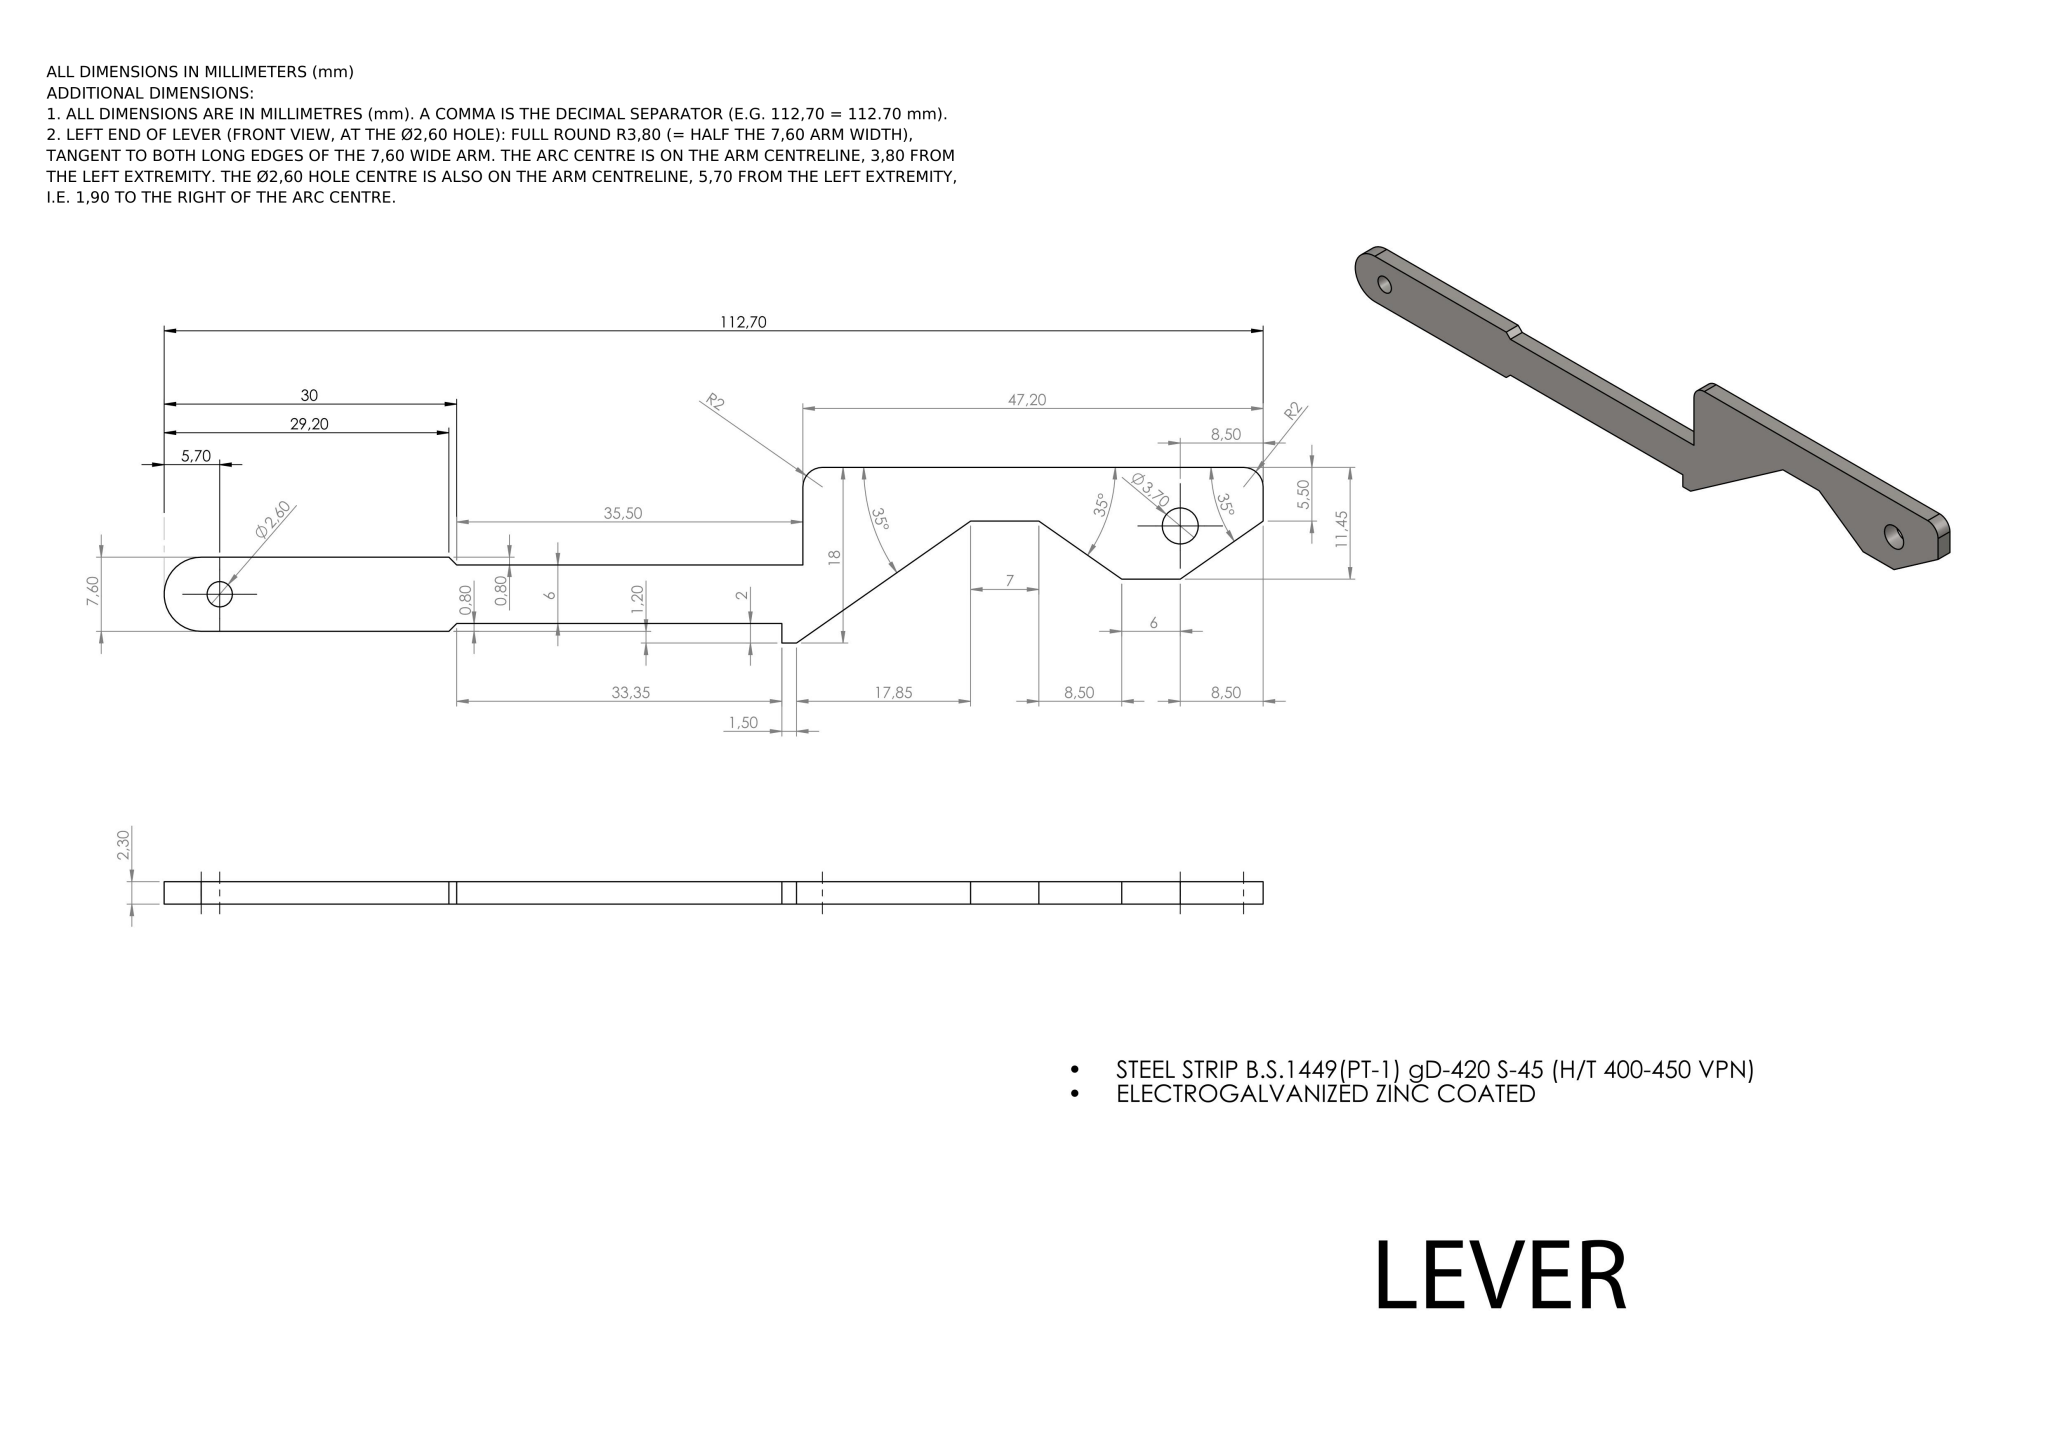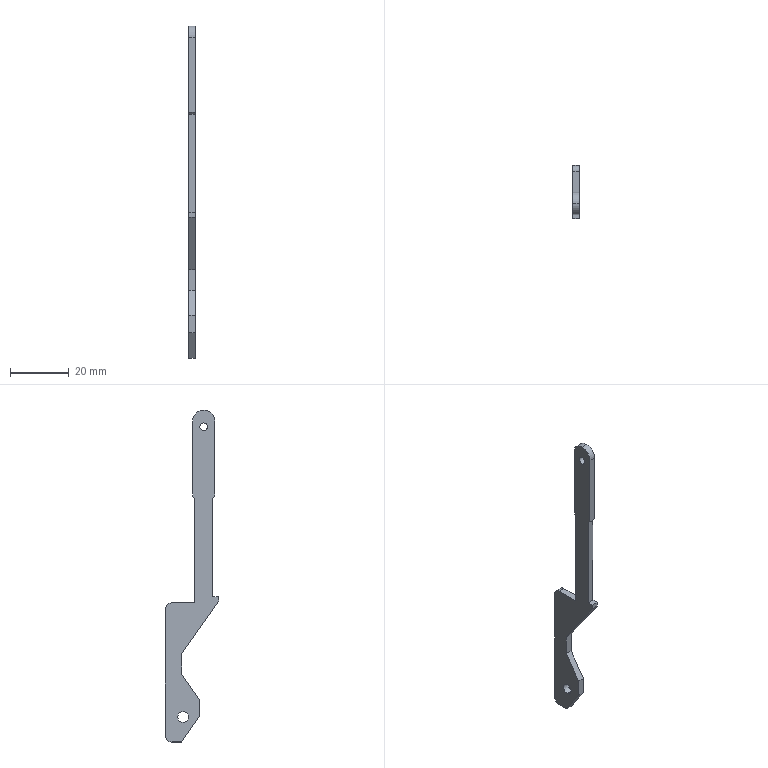Part | NX | mm | Stepped Dual-Ear Link Bracket | 1 solid | 26 faces | box 2.3 x 18 x 112.7 mm | volume 2001 mm3 | plane 18 | cylinder 8 | commonest cylinder face diameters 3.7 x2 2.6 x2 7.6 x2 4 x2